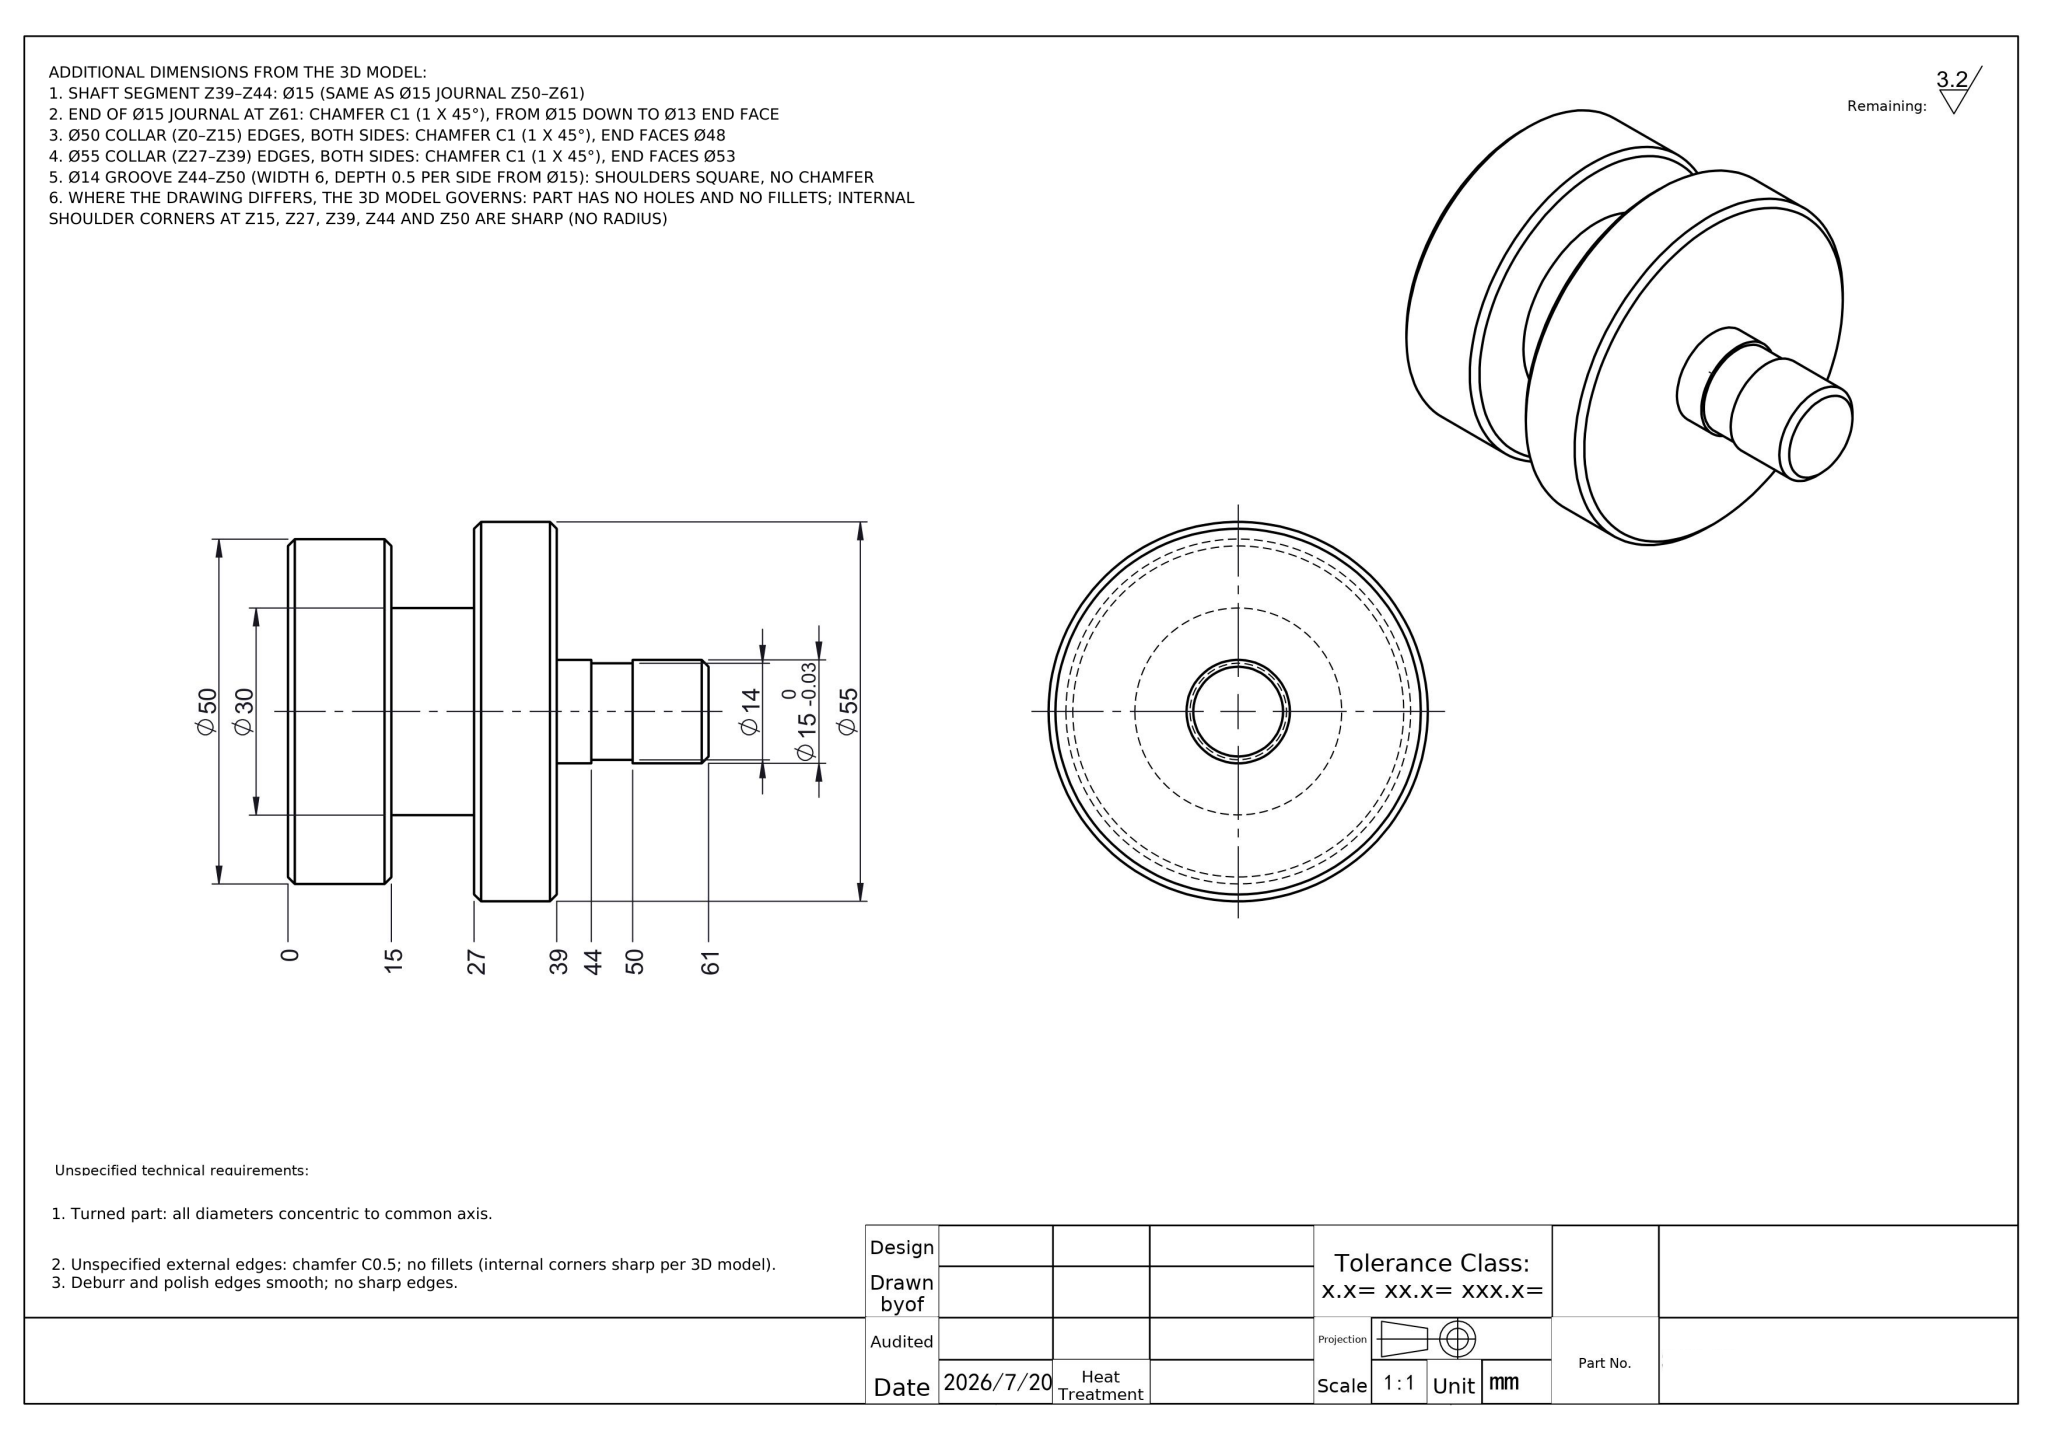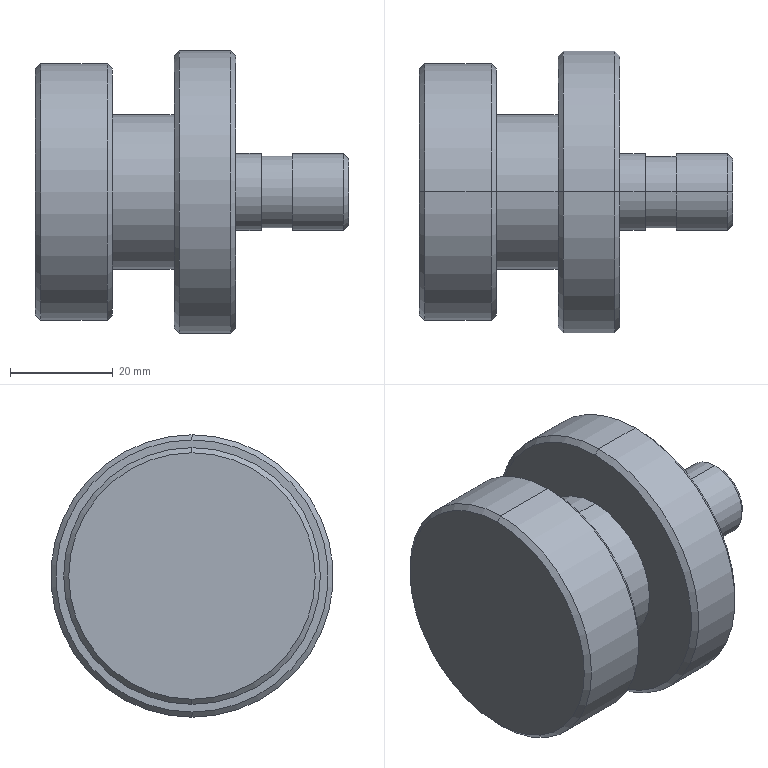Part | NX | mm | 1 solid | 29 faces | box 61 x 55 x 55 mm | volume 69848 mm3 | cylinder 12 | cone 10 | plane 7 | commonest cylinder face diameters 15 x4 14 x2 50 x2 30 x2 55 x2
STEP:
#1=CARTESIAN_POINT('',(39.,0.,-26.5));
#2=VERTEX_POINT('',#1);
#3=CARTESIAN_POINT('',(39.,0.,26.5));
#4=VERTEX_POINT('',#3);
#5=CARTESIAN_POINT('',(39.,0.,0.));
#6=DIRECTION('',(1.,0.,0.));
#7=DIRECTION('',(0.,0.,1.));
#8=AXIS2_PLACEMENT_3D('',#5,#6,#7);
#9=CIRCLE('',#8,26.5);
#10=EDGE_CURVE('',#2,#4,#9,.T.);
#11=ORIENTED_EDGE('',*,*,#10,.F.);
#12=CARTESIAN_POINT('',(38.,0.,-27.5));
#13=VERTEX_POINT('',#12);
#14=CARTESIAN_POINT('',(38.,0.,-27.5));
#15=DIRECTION('',(-0.7071,0.,-0.7071));
#16=VECTOR('',#15,1000.);
#17=LINE('',#14,#16);
#18=EDGE_CURVE('',#2,#13,#17,.T.);
#19=ORIENTED_EDGE('',*,*,#18,.T.);
#20=CARTESIAN_POINT('',(38.,0.,27.5));
#21=VERTEX_POINT('',#20);
#22=CARTESIAN_POINT('',(38.,0.,0.));
#23=DIRECTION('',(-1.,0.,0.));
#24=DIRECTION('',(0.,0.,1.));
#25=AXIS2_PLACEMENT_3D('',#22,#23,#24);
#26=CIRCLE('',#25,27.5);
#27=EDGE_CURVE('',#21,#13,#26,.T.);
#28=ORIENTED_EDGE('',*,*,#27,.F.);
#29=CARTESIAN_POINT('',(38.,0.,27.5));
#30=DIRECTION('',(-0.7071,0.,0.7071));
#31=VECTOR('',#30,1000.);
#32=LINE('',#29,#31);
#33=EDGE_CURVE('',#4,#21,#32,.T.);
#34=ORIENTED_EDGE('',*,*,#33,.F.);
#35=EDGE_LOOP('',(#11,#19,#28,#34));
#36=FACE_OUTER_BOUND('',#35,.T.);
#37=CARTESIAN_POINT('',(38.,0.,0.));
#38=DIRECTION('',(-1.,0.,0.));
#39=DIRECTION('',(0.,0.,1.));
#40=AXIS2_PLACEMENT_3D('',#37,#38,#39);
#41=CONICAL_SURFACE('',#40,27.5,0.7854);
#42=ADVANCED_FACE('',(#36),#41,.T.);
#43=CARTESIAN_POINT('',(61.,0.,-6.5));
#44=VERTEX_POINT('',#43);
#45=CARTESIAN_POINT('',(61.,0.,6.5));
#46=VERTEX_POINT('',#45);
#47=CARTESIAN_POINT('',(61.,0.,0.));
#48=DIRECTION('',(1.,0.,0.));
#49=DIRECTION('',(0.,0.,-1.));
#50=AXIS2_PLACEMENT_3D('',#47,#48,#49);
#51=CIRCLE('',#50,6.5);
#52=EDGE_CURVE('',#44,#46,#51,.T.);
#53=ORIENTED_EDGE('',*,*,#52,.F.);
#54=CARTESIAN_POINT('',(60.,0.,-7.5));
#55=VERTEX_POINT('',#54);
#56=CARTESIAN_POINT('',(61.,0.,-6.5));
#57=DIRECTION('',(-0.7071,0.,-0.7071));
#58=VECTOR('',#57,1000.);
#59=LINE('',#56,#58);
#60=EDGE_CURVE('',#44,#55,#59,.T.);
#61=ORIENTED_EDGE('',*,*,#60,.T.);
#62=CARTESIAN_POINT('',(60.,0.,7.5));
#63=VERTEX_POINT('',#62);
#64=CARTESIAN_POINT('',(60.,0.,0.));
#65=DIRECTION('',(-1.,0.,0.));
#66=DIRECTION('',(0.,0.,-1.));
#67=AXIS2_PLACEMENT_3D('',#64,#65,#66);
#68=CIRCLE('',#67,7.5);
#69=EDGE_CURVE('',#63,#55,#68,.T.);
#70=ORIENTED_EDGE('',*,*,#69,.F.);
#71=CARTESIAN_POINT('',(61.,0.,6.5));
#72=DIRECTION('',(-0.7071,0.,0.7071));
#73=VECTOR('',#72,1000.);
#74=LINE('',#71,#73);
#75=EDGE_CURVE('',#46,#63,#74,.T.);
#76=ORIENTED_EDGE('',*,*,#75,.F.);
#77=EDGE_LOOP('',(#53,#61,#70,#76));
#78=FACE_OUTER_BOUND('',#77,.T.);
#79=CARTESIAN_POINT('',(61.,0.,0.));
#80=DIRECTION('',(-1.,0.,0.));
#81=DIRECTION('',(0.,0.,1.));
#82=AXIS2_PLACEMENT_3D('',#79,#80,#81);
#83=CONICAL_SURFACE('',#82,6.5,0.7854);
#84=ADVANCED_FACE('',(#78),#83,.T.);
#85=ORIENTED_EDGE('',*,*,#69,.T.);
#86=CARTESIAN_POINT('',(50.,0.,-7.5));
#87=VERTEX_POINT('',#86);
#88=CARTESIAN_POINT('',(61.,0.,-7.5));
#89=DIRECTION('',(-1.,0.,0.));
#90=VECTOR('',#89,1000.);
#91=LINE('',#88,#90);
#92=EDGE_CURVE('',#55,#87,#91,.T.);
#93=ORIENTED_EDGE('',*,*,#92,.T.);
#94=CARTESIAN_POINT('',(50.,0.,7.5));
#95=VERTEX_POINT('',#94);
#96=CARTESIAN_POINT('',(50.,0.,0.));
#97=DIRECTION('',(1.,0.,0.));
#98=DIRECTION('',(0.,0.,-1.));
#99=AXIS2_PLACEMENT_3D('',#96,#97,#98);
#100=CIRCLE('',#99,7.5);
#101=EDGE_CURVE('',#87,#95,#100,.T.);
#102=ORIENTED_EDGE('',*,*,#101,.T.);
#103=CARTESIAN_POINT('',(61.,0.,7.5));
#104=DIRECTION('',(-1.,0.,0.));
#105=VECTOR('',#104,1000.);
#106=LINE('',#103,#105);
#107=EDGE_CURVE('',#63,#95,#106,.T.);
#108=ORIENTED_EDGE('',*,*,#107,.F.);
#109=EDGE_LOOP('',(#85,#93,#102,#108));
#110=FACE_OUTER_BOUND('',#109,.T.);
#111=CARTESIAN_POINT('',(61.,0.,0.));
#112=DIRECTION('',(-1.,0.,0.));
#113=DIRECTION('',(0.,0.,1.));
#114=AXIS2_PLACEMENT_3D('',#111,#112,#113);
#115=CYLINDRICAL_SURFACE('',#114,7.5);
#116=ADVANCED_FACE('',(#110),#115,.T.);
#117=CARTESIAN_POINT('',(50.,0.,-7.));
#118=VERTEX_POINT('',#117);
#119=CARTESIAN_POINT('',(50.,0.,7.));
#120=VERTEX_POINT('',#119);
#121=CARTESIAN_POINT('',(50.,0.,0.));
#122=DIRECTION('',(1.,0.,0.));
#123=DIRECTION('',(0.,0.,-1.));
#124=AXIS2_PLACEMENT_3D('',#121,#122,#123);
#125=CIRCLE('',#124,7.);
#126=EDGE_CURVE('',#118,#120,#125,.T.);
#127=ORIENTED_EDGE('',*,*,#126,.F.);
#128=CARTESIAN_POINT('',(44.,0.,-7.));
#129=VERTEX_POINT('',#128);
#130=CARTESIAN_POINT('',(50.,0.,-7.));
#131=DIRECTION('',(-1.,0.,0.));
#132=VECTOR('',#131,1000.);
#133=LINE('',#130,#132);
#134=EDGE_CURVE('',#118,#129,#133,.T.);
#135=ORIENTED_EDGE('',*,*,#134,.T.);
#136=CARTESIAN_POINT('',(44.,0.,7.));
#137=VERTEX_POINT('',#136);
#138=CARTESIAN_POINT('',(44.,0.,0.));
#139=DIRECTION('',(1.,0.,0.));
#140=DIRECTION('',(0.,0.,-1.));
#141=AXIS2_PLACEMENT_3D('',#138,#139,#140);
#142=CIRCLE('',#141,7.);
#143=EDGE_CURVE('',#129,#137,#142,.T.);
#144=ORIENTED_EDGE('',*,*,#143,.T.);
#145=CARTESIAN_POINT('',(50.,0.,7.));
#146=DIRECTION('',(-1.,0.,0.));
#147=VECTOR('',#146,1000.);
#148=LINE('',#145,#147);
#149=EDGE_CURVE('',#120,#137,#148,.T.);
#150=ORIENTED_EDGE('',*,*,#149,.F.);
#151=EDGE_LOOP('',(#127,#135,#144,#150));
#152=FACE_OUTER_BOUND('',#151,.T.);
#153=CARTESIAN_POINT('',(50.,0.,0.));
#154=DIRECTION('',(-1.,0.,0.));
#155=DIRECTION('',(0.,0.,1.));
#156=AXIS2_PLACEMENT_3D('',#153,#154,#155);
#157=CYLINDRICAL_SURFACE('',#156,7.);
#158=ADVANCED_FACE('',(#152),#157,.T.);
#159=CARTESIAN_POINT('',(27.,0.,26.5));
#160=VERTEX_POINT('',#159);
#161=CARTESIAN_POINT('',(27.,0.,-26.5));
#162=VERTEX_POINT('',#161);
#163=CARTESIAN_POINT('',(27.,0.,0.));
#164=DIRECTION('',(-1.,0.,0.));
#165=DIRECTION('',(0.,0.,-1.));
#166=AXIS2_PLACEMENT_3D('',#163,#164,#165);
#167=CIRCLE('',#166,26.5);
#168=EDGE_CURVE('',#160,#162,#167,.T.);
#169=ORIENTED_EDGE('',*,*,#168,.F.);
#170=CARTESIAN_POINT('',(28.,0.,27.5));
#171=VERTEX_POINT('',#170);
#172=CARTESIAN_POINT('',(27.,0.,26.5));
#173=DIRECTION('',(0.7071,0.,0.7071));
#174=VECTOR('',#173,1000.);
#175=LINE('',#172,#174);
#176=EDGE_CURVE('',#160,#171,#175,.T.);
#177=ORIENTED_EDGE('',*,*,#176,.T.);
#178=CARTESIAN_POINT('',(28.,0.,-27.5));
#179=VERTEX_POINT('',#178);
#180=CARTESIAN_POINT('',(28.,0.,0.));
#181=DIRECTION('',(1.,0.,0.));
#182=DIRECTION('',(0.,0.,-1.));
#183=AXIS2_PLACEMENT_3D('',#180,#181,#182);
#184=CIRCLE('',#183,27.5);
#185=EDGE_CURVE('',#179,#171,#184,.T.);
#186=ORIENTED_EDGE('',*,*,#185,.F.);
#187=CARTESIAN_POINT('',(27.,0.,-26.5));
#188=DIRECTION('',(0.7071,0.,-0.7071));
#189=VECTOR('',#188,1000.);
#190=LINE('',#187,#189);
#191=EDGE_CURVE('',#162,#179,#190,.T.);
#192=ORIENTED_EDGE('',*,*,#191,.F.);
#193=EDGE_LOOP('',(#169,#177,#186,#192));
#194=FACE_OUTER_BOUND('',#193,.T.);
#195=CARTESIAN_POINT('',(27.,0.,0.));
#196=DIRECTION('',(1.,0.,0.));
#197=DIRECTION('',(0.,0.,-1.));
#198=AXIS2_PLACEMENT_3D('',#195,#196,#197);
#199=CONICAL_SURFACE('',#198,26.5,0.7854);
#200=ADVANCED_FACE('',(#194),#199,.T.);
#201=CARTESIAN_POINT('',(-0.,0.,24.));
#202=VERTEX_POINT('',#201);
#203=CARTESIAN_POINT('',(-0.,0.,-24.));
#204=VERTEX_POINT('',#203);
#205=CARTESIAN_POINT('',(-0.,0.,0.));
#206=DIRECTION('',(-1.,0.,0.));
#207=DIRECTION('',(0.,0.,-1.));
#208=AXIS2_PLACEMENT_3D('',#205,#206,#207);
#209=CIRCLE('',#208,24.);
#210=EDGE_CURVE('',#202,#204,#209,.T.);
#211=ORIENTED_EDGE('',*,*,#210,.F.);
#212=CARTESIAN_POINT('',(1.,0.,25.));
#213=VERTEX_POINT('',#212);
#214=CARTESIAN_POINT('',(-0.,0.,24.));
#215=DIRECTION('',(0.7071,0.,0.7071));
#216=VECTOR('',#215,1000.);
#217=LINE('',#214,#216);
#218=EDGE_CURVE('',#202,#213,#217,.T.);
#219=ORIENTED_EDGE('',*,*,#218,.T.);
#220=CARTESIAN_POINT('',(1.,0.,-25.));
#221=VERTEX_POINT('',#220);
#222=CARTESIAN_POINT('',(1.,0.,0.));
#223=DIRECTION('',(1.,0.,0.));
#224=DIRECTION('',(0.,0.,-1.));
#225=AXIS2_PLACEMENT_3D('',#222,#223,#224);
#226=CIRCLE('',#225,25.);
#227=EDGE_CURVE('',#221,#213,#226,.T.);
#228=ORIENTED_EDGE('',*,*,#227,.F.);
#229=CARTESIAN_POINT('',(-0.,0.,-24.));
#230=DIRECTION('',(0.7071,0.,-0.7071));
#231=VECTOR('',#230,1000.);
#232=LINE('',#229,#231);
#233=EDGE_CURVE('',#204,#221,#232,.T.);
#234=ORIENTED_EDGE('',*,*,#233,.F.);
#235=EDGE_LOOP('',(#211,#219,#228,#234));
#236=FACE_OUTER_BOUND('',#235,.T.);
#237=CARTESIAN_POINT('',(-0.,0.,0.));
#238=DIRECTION('',(1.,0.,0.));
#239=DIRECTION('',(0.,0.,-1.));
#240=AXIS2_PLACEMENT_3D('',#237,#238,#239);
#241=CONICAL_SURFACE('',#240,24.,0.7854);
#242=ADVANCED_FACE('',(#236),#241,.T.);
#243=CARTESIAN_POINT('',(15.,0.,-24.));
#244=VERTEX_POINT('',#243);
#245=CARTESIAN_POINT('',(15.,0.,24.));
#246=VERTEX_POINT('',#245);
#247=CARTESIAN_POINT('',(15.,0.,0.));
#248=DIRECTION('',(1.,0.,0.));
#249=DIRECTION('',(0.,0.,1.));
#250=AXIS2_PLACEMENT_3D('',#247,#248,#249);
#251=CIRCLE('',#250,24.);
#252=EDGE_CURVE('',#244,#246,#251,.T.);
#253=ORIENTED_EDGE('',*,*,#252,.F.);
#254=CARTESIAN_POINT('',(14.,0.,-25.));
#255=VERTEX_POINT('',#254);
#256=CARTESIAN_POINT('',(14.,0.,-25.));
#257=DIRECTION('',(-0.7071,0.,-0.7071));
#258=VECTOR('',#257,1000.);
#259=LINE('',#256,#258);
#260=EDGE_CURVE('',#244,#255,#259,.T.);
#261=ORIENTED_EDGE('',*,*,#260,.T.);
#262=CARTESIAN_POINT('',(14.,0.,25.));
#263=VERTEX_POINT('',#262);
#264=CARTESIAN_POINT('',(14.,0.,0.));
#265=DIRECTION('',(-1.,0.,0.));
#266=DIRECTION('',(0.,0.,1.));
#267=AXIS2_PLACEMENT_3D('',#264,#265,#266);
#268=CIRCLE('',#267,25.);
#269=EDGE_CURVE('',#263,#255,#268,.T.);
#270=ORIENTED_EDGE('',*,*,#269,.F.);
#271=CARTESIAN_POINT('',(14.,0.,25.));
#272=DIRECTION('',(-0.7071,0.,0.7071));
#273=VECTOR('',#272,1000.);
#274=LINE('',#271,#273);
#275=EDGE_CURVE('',#246,#263,#274,.T.);
#276=ORIENTED_EDGE('',*,*,#275,.F.);
#277=EDGE_LOOP('',(#253,#261,#270,#276));
#278=FACE_OUTER_BOUND('',#277,.T.);
#279=CARTESIAN_POINT('',(14.,0.,0.));
#280=DIRECTION('',(-1.,0.,0.));
#281=DIRECTION('',(0.,0.,1.));
#282=AXIS2_PLACEMENT_3D('',#279,#280,#281);
#283=CONICAL_SURFACE('',#282,25.,0.7854);
#284=ADVANCED_FACE('',(#278),#283,.T.);
#285=ORIENTED_EDGE('',*,*,#269,.T.);
#286=CARTESIAN_POINT('',(0.,0.,-25.));
#287=DIRECTION('',(-1.,0.,0.));
#288=VECTOR('',#287,1000.);
#289=LINE('',#286,#288);
#290=EDGE_CURVE('',#255,#221,#289,.T.);
#291=ORIENTED_EDGE('',*,*,#290,.T.);
#292=ORIENTED_EDGE('',*,*,#227,.T.);
#293=CARTESIAN_POINT('',(0.,0.,25.));
#294=DIRECTION('',(-1.,0.,0.));
#295=VECTOR('',#294,1000.);
#296=LINE('',#293,#295);
#297=EDGE_CURVE('',#263,#213,#296,.T.);
#298=ORIENTED_EDGE('',*,*,#297,.F.);
#299=EDGE_LOOP('',(#285,#291,#292,#298));
#300=FACE_OUTER_BOUND('',#299,.T.);
#301=CARTESIAN_POINT('',(0.,0.,0.));
#302=DIRECTION('',(-1.,0.,0.));
#303=DIRECTION('',(0.,0.,1.));
#304=AXIS2_PLACEMENT_3D('',#301,#302,#303);
#305=CYLINDRICAL_SURFACE('',#304,25.);
#306=ADVANCED_FACE('',(#300),#305,.T.);
#307=CARTESIAN_POINT('',(27.,0.,15.));
#308=VERTEX_POINT('',#307);
#309=CARTESIAN_POINT('',(27.,0.,-15.));
#310=VERTEX_POINT('',#309);
#311=CARTESIAN_POINT('',(27.,0.,0.));
#312=DIRECTION('',(-1.,0.,0.));
#313=DIRECTION('',(0.,0.,1.));
#314=AXIS2_PLACEMENT_3D('',#311,#312,#313);
#315=CIRCLE('',#314,15.);
#316=EDGE_CURVE('',#308,#310,#315,.T.);
#317=ORIENTED_EDGE('',*,*,#316,.T.);
#318=CARTESIAN_POINT('',(15.,0.,-15.));
#319=VERTEX_POINT('',#318);
#320=CARTESIAN_POINT('',(0.,0.,-15.));
#321=DIRECTION('',(-1.,0.,0.));
#322=VECTOR('',#321,1000.);
#323=LINE('',#320,#322);
#324=EDGE_CURVE('',#310,#319,#323,.T.);
#325=ORIENTED_EDGE('',*,*,#324,.T.);
#326=CARTESIAN_POINT('',(15.,0.,15.));
#327=VERTEX_POINT('',#326);
#328=CARTESIAN_POINT('',(15.,0.,0.));
#329=DIRECTION('',(-1.,0.,0.));
#330=DIRECTION('',(0.,0.,1.));
#331=AXIS2_PLACEMENT_3D('',#328,#329,#330);
#332=CIRCLE('',#331,15.);
#333=EDGE_CURVE('',#327,#319,#332,.T.);
#334=ORIENTED_EDGE('',*,*,#333,.F.);
#335=CARTESIAN_POINT('',(0.,0.,15.));
#336=DIRECTION('',(-1.,0.,0.));
#337=VECTOR('',#336,1000.);
#338=LINE('',#335,#337);
#339=EDGE_CURVE('',#308,#327,#338,.T.);
#340=ORIENTED_EDGE('',*,*,#339,.F.);
#341=EDGE_LOOP('',(#317,#325,#334,#340));
#342=FACE_OUTER_BOUND('',#341,.T.);
#343=CARTESIAN_POINT('',(0.,0.,0.));
#344=DIRECTION('',(-1.,0.,0.));
#345=DIRECTION('',(0.,0.,1.));
#346=AXIS2_PLACEMENT_3D('',#343,#344,#345);
#347=CYLINDRICAL_SURFACE('',#346,15.);
#348=ADVANCED_FACE('',(#342),#347,.T.);
#349=ORIENTED_EDGE('',*,*,#27,.T.);
#350=CARTESIAN_POINT('',(0.,0.,-27.5));
#351=DIRECTION('',(-1.,0.,0.));
#352=VECTOR('',#351,1000.);
#353=LINE('',#350,#352);
#354=EDGE_CURVE('',#13,#179,#353,.T.);
#355=ORIENTED_EDGE('',*,*,#354,.T.);
#356=ORIENTED_EDGE('',*,*,#185,.T.);
#357=CARTESIAN_POINT('',(0.,0.,27.5));
#358=DIRECTION('',(-1.,0.,0.));
#359=VECTOR('',#358,1000.);
#360=LINE('',#357,#359);
#361=EDGE_CURVE('',#21,#171,#360,.T.);
#362=ORIENTED_EDGE('',*,*,#361,.F.);
#363=EDGE_LOOP('',(#349,#355,#356,#362));
#364=FACE_OUTER_BOUND('',#363,.T.);
#365=CARTESIAN_POINT('',(0.,0.,0.));
#366=DIRECTION('',(-1.,0.,0.));
#367=DIRECTION('',(0.,0.,1.));
#368=AXIS2_PLACEMENT_3D('',#365,#366,#367);
#369=CYLINDRICAL_SURFACE('',#368,27.5);
#370=ADVANCED_FACE('',(#364),#369,.T.);
#371=CARTESIAN_POINT('',(44.,0.,-7.5));
#372=VERTEX_POINT('',#371);
#373=CARTESIAN_POINT('',(44.,0.,7.5));
#374=VERTEX_POINT('',#373);
#375=CARTESIAN_POINT('',(44.,0.,0.));
#376=DIRECTION('',(1.,0.,0.));
#377=DIRECTION('',(0.,0.,-1.));
#378=AXIS2_PLACEMENT_3D('',#375,#376,#377);
#379=CIRCLE('',#378,7.5);
#380=EDGE_CURVE('',#372,#374,#379,.T.);
#381=ORIENTED_EDGE('',*,*,#380,.F.);
#382=CARTESIAN_POINT('',(39.,0.,-7.5));
#383=VERTEX_POINT('',#382);
#384=CARTESIAN_POINT('',(61.,0.,-7.5));
#385=DIRECTION('',(-1.,0.,0.));
#386=VECTOR('',#385,1000.);
#387=LINE('',#384,#386);
#388=EDGE_CURVE('',#372,#383,#387,.T.);
#389=ORIENTED_EDGE('',*,*,#388,.T.);
#390=CARTESIAN_POINT('',(39.,0.,7.5));
#391=VERTEX_POINT('',#390);
#392=CARTESIAN_POINT('',(39.,0.,0.));
#393=DIRECTION('',(1.,0.,0.));
#394=DIRECTION('',(0.,0.,1.));
#395=AXIS2_PLACEMENT_3D('',#392,#393,#394);
#396=CIRCLE('',#395,7.5);
#397=EDGE_CURVE('',#383,#391,#396,.T.);
#398=ORIENTED_EDGE('',*,*,#397,.T.);
#399=CARTESIAN_POINT('',(61.,0.,7.5));
#400=DIRECTION('',(-1.,0.,0.));
#401=VECTOR('',#400,1000.);
#402=LINE('',#399,#401);
#403=EDGE_CURVE('',#374,#391,#402,.T.);
#404=ORIENTED_EDGE('',*,*,#403,.F.);
#405=EDGE_LOOP('',(#381,#389,#398,#404));
#406=FACE_OUTER_BOUND('',#405,.T.);
#407=CARTESIAN_POINT('',(61.,0.,0.));
#408=DIRECTION('',(-1.,0.,0.));
#409=DIRECTION('',(0.,0.,1.));
#410=AXIS2_PLACEMENT_3D('',#407,#408,#409);
#411=CYLINDRICAL_SURFACE('',#410,7.5);
#412=ADVANCED_FACE('',(#406),#411,.T.);
#413=ORIENTED_EDGE('',*,*,#388,.F.);
#414=CARTESIAN_POINT('',(44.,0.,0.));
#415=DIRECTION('',(1.,0.,0.));
#416=DIRECTION('',(0.,0.,-1.));
#417=AXIS2_PLACEMENT_3D('',#414,#415,#416);
#418=CIRCLE('',#417,7.5);
#419=EDGE_CURVE('',#374,#372,#418,.T.);
#420=ORIENTED_EDGE('',*,*,#419,.F.);
#421=ORIENTED_EDGE('',*,*,#403,.T.);
#422=CARTESIAN_POINT('',(39.,0.,0.));
#423=DIRECTION('',(1.,0.,0.));
#424=DIRECTION('',(0.,0.,1.));
#425=AXIS2_PLACEMENT_3D('',#422,#423,#424);
#426=CIRCLE('',#425,7.5);
#427=EDGE_CURVE('',#391,#383,#426,.T.);
#428=ORIENTED_EDGE('',*,*,#427,.T.);
#429=EDGE_LOOP('',(#413,#420,#421,#428));
#430=FACE_OUTER_BOUND('',#429,.T.);
#431=CARTESIAN_POINT('',(61.,0.,0.));
#432=DIRECTION('',(-1.,0.,0.));
#433=DIRECTION('',(0.,0.,1.));
#434=AXIS2_PLACEMENT_3D('',#431,#432,#433);
#435=CYLINDRICAL_SURFACE('',#434,7.5);
#436=ADVANCED_FACE('',(#430),#435,.T.);
#437=CARTESIAN_POINT('',(39.,0.,0.));
#438=DIRECTION('',(1.,0.,0.));
#439=DIRECTION('',(0.,0.,1.));
#440=AXIS2_PLACEMENT_3D('',#437,#438,#439);
#441=CIRCLE('',#440,26.5);
#442=EDGE_CURVE('',#4,#2,#441,.T.);
#443=ORIENTED_EDGE('',*,*,#442,.T.);
#444=ORIENTED_EDGE('',*,*,#10,.T.);
#445=EDGE_LOOP('',(#443,#444));
#446=FACE_OUTER_BOUND('',#445,.T.);
#447=ORIENTED_EDGE('',*,*,#427,.F.);
#448=ORIENTED_EDGE('',*,*,#397,.F.);
#449=EDGE_LOOP('',(#447,#448));
#450=FACE_BOUND('',#449,.T.);
#451=CARTESIAN_POINT('',(39.,0.,0.));
#452=DIRECTION('',(-1.,0.,0.));
#453=DIRECTION('',(0.,0.,1.));
#454=AXIS2_PLACEMENT_3D('',#451,#452,#453);
#455=PLANE('',#454);
#456=ADVANCED_FACE('',(#446,#450),#455,.F.);
#457=CARTESIAN_POINT('',(-0.,0.,0.));
#458=DIRECTION('',(-1.,0.,0.));
#459=DIRECTION('',(0.,0.,-1.));
#460=AXIS2_PLACEMENT_3D('',#457,#458,#459);
#461=CIRCLE('',#460,24.);
#462=EDGE_CURVE('',#204,#202,#461,.T.);
#463=ORIENTED_EDGE('',*,*,#462,.T.);
#464=ORIENTED_EDGE('',*,*,#210,.T.);
#465=EDGE_LOOP('',(#463,#464));
#466=FACE_OUTER_BOUND('',#465,.T.);
#467=CARTESIAN_POINT('',(-0.,25.,0.));
#468=DIRECTION('',(1.,0.,0.));
#469=DIRECTION('',(0.,0.,-1.));
#470=AXIS2_PLACEMENT_3D('',#467,#468,#469);
#471=PLANE('',#470);
#472=ADVANCED_FACE('',(#466),#471,.F.);
#473=ORIENTED_EDGE('',*,*,#354,.F.);
#474=CARTESIAN_POINT('',(38.,0.,0.));
#475=DIRECTION('',(-1.,0.,0.));
#476=DIRECTION('',(0.,0.,1.));
#477=AXIS2_PLACEMENT_3D('',#474,#475,#476);
#478=CIRCLE('',#477,27.5);
#479=EDGE_CURVE('',#13,#21,#478,.T.);
#480=ORIENTED_EDGE('',*,*,#479,.T.);
#481=ORIENTED_EDGE('',*,*,#361,.T.);
#482=CARTESIAN_POINT('',(28.,0.,0.));
#483=DIRECTION('',(1.,0.,0.));
#484=DIRECTION('',(0.,0.,-1.));
#485=AXIS2_PLACEMENT_3D('',#482,#483,#484);
#486=CIRCLE('',#485,27.5);
#487=EDGE_CURVE('',#171,#179,#486,.T.);
#488=ORIENTED_EDGE('',*,*,#487,.T.);
#489=EDGE_LOOP('',(#473,#480,#481,#488));
#490=FACE_OUTER_BOUND('',#489,.T.);
#491=CARTESIAN_POINT('',(0.,0.,0.));
#492=DIRECTION('',(-1.,0.,0.));
#493=DIRECTION('',(0.,0.,1.));
#494=AXIS2_PLACEMENT_3D('',#491,#492,#493);
#495=CYLINDRICAL_SURFACE('',#494,27.5);
#496=ADVANCED_FACE('',(#490),#495,.T.);
#497=CARTESIAN_POINT('',(27.,0.,0.));
#498=DIRECTION('',(-1.,0.,0.));
#499=DIRECTION('',(0.,0.,-1.));
#500=AXIS2_PLACEMENT_3D('',#497,#498,#499);
#501=CIRCLE('',#500,26.5);
#502=EDGE_CURVE('',#162,#160,#501,.T.);
#503=ORIENTED_EDGE('',*,*,#502,.T.);
#504=ORIENTED_EDGE('',*,*,#168,.T.);
#505=EDGE_LOOP('',(#503,#504));
#506=FACE_OUTER_BOUND('',#505,.T.);
#507=ORIENTED_EDGE('',*,*,#316,.F.);
#508=CARTESIAN_POINT('',(27.,0.,0.));
#509=DIRECTION('',(-1.,0.,0.));
#510=DIRECTION('',(0.,0.,1.));
#511=AXIS2_PLACEMENT_3D('',#508,#509,#510);
#512=CIRCLE('',#511,15.);
#513=EDGE_CURVE('',#310,#308,#512,.T.);
#514=ORIENTED_EDGE('',*,*,#513,.F.);
#515=EDGE_LOOP('',(#507,#514));
#516=FACE_BOUND('',#515,.T.);
#517=CARTESIAN_POINT('',(27.,27.5,0.));
#518=DIRECTION('',(1.,0.,0.));
#519=DIRECTION('',(0.,0.,-1.));
#520=AXIS2_PLACEMENT_3D('',#517,#518,#519);
#521=PLANE('',#520);
#522=ADVANCED_FACE('',(#506,#516),#521,.F.);
#523=ORIENTED_EDGE('',*,*,#324,.F.);
#524=ORIENTED_EDGE('',*,*,#513,.T.);
#525=ORIENTED_EDGE('',*,*,#339,.T.);
#526=CARTESIAN_POINT('',(15.,0.,0.));
#527=DIRECTION('',(-1.,0.,0.));
#528=DIRECTION('',(0.,0.,1.));
#529=AXIS2_PLACEMENT_3D('',#526,#527,#528);
#530=CIRCLE('',#529,15.);
#531=EDGE_CURVE('',#319,#327,#530,.T.);
#532=ORIENTED_EDGE('',*,*,#531,.F.);
#533=EDGE_LOOP('',(#523,#524,#525,#532));
#534=FACE_OUTER_BOUND('',#533,.T.);
#535=CARTESIAN_POINT('',(0.,0.,0.));
#536=DIRECTION('',(-1.,0.,0.));
#537=DIRECTION('',(0.,0.,1.));
#538=AXIS2_PLACEMENT_3D('',#535,#536,#537);
#539=CYLINDRICAL_SURFACE('',#538,15.);
#540=ADVANCED_FACE('',(#534),#539,.T.);
#541=CARTESIAN_POINT('',(15.,0.,0.));
#542=DIRECTION('',(1.,0.,0.));
#543=DIRECTION('',(0.,0.,1.));
#544=AXIS2_PLACEMENT_3D('',#541,#542,#543);
#545=CIRCLE('',#544,24.);
#546=EDGE_CURVE('',#246,#244,#545,.T.);
#547=ORIENTED_EDGE('',*,*,#546,.T.);
#548=ORIENTED_EDGE('',*,*,#252,.T.);
#549=EDGE_LOOP('',(#547,#548));
#550=FACE_OUTER_BOUND('',#549,.T.);
#551=ORIENTED_EDGE('',*,*,#333,.T.);
#552=ORIENTED_EDGE('',*,*,#531,.T.);
#553=EDGE_LOOP('',(#551,#552));
#554=FACE_BOUND('',#553,.T.);
#555=CARTESIAN_POINT('',(15.,15.,0.));
#556=DIRECTION('',(-1.,0.,0.));
#557=DIRECTION('',(0.,0.,1.));
#558=AXIS2_PLACEMENT_3D('',#555,#556,#557);
#559=PLANE('',#558);
#560=ADVANCED_FACE('',(#550,#554),#559,.F.);
#561=ORIENTED_EDGE('',*,*,#290,.F.);
#562=CARTESIAN_POINT('',(14.,0.,0.));
#563=DIRECTION('',(-1.,0.,0.));
#564=DIRECTION('',(0.,0.,1.));
#565=AXIS2_PLACEMENT_3D('',#562,#563,#564);
#566=CIRCLE('',#565,25.);
#567=EDGE_CURVE('',#255,#263,#566,.T.);
#568=ORIENTED_EDGE('',*,*,#567,.T.);
#569=ORIENTED_EDGE('',*,*,#297,.T.);
#570=CARTESIAN_POINT('',(1.,0.,0.));
#571=DIRECTION('',(1.,0.,0.));
#572=DIRECTION('',(0.,0.,-1.));
#573=AXIS2_PLACEMENT_3D('',#570,#571,#572);
#574=CIRCLE('',#573,25.);
#575=EDGE_CURVE('',#213,#221,#574,.T.);
#576=ORIENTED_EDGE('',*,*,#575,.T.);
#577=EDGE_LOOP('',(#561,#568,#569,#576));
#578=FACE_OUTER_BOUND('',#577,.T.);
#579=CARTESIAN_POINT('',(0.,0.,0.));
#580=DIRECTION('',(-1.,0.,0.));
#581=DIRECTION('',(0.,0.,1.));
#582=AXIS2_PLACEMENT_3D('',#579,#580,#581);
#583=CYLINDRICAL_SURFACE('',#582,25.);
#584=ADVANCED_FACE('',(#578),#583,.T.);
#585=ORIENTED_EDGE('',*,*,#260,.F.);
#586=ORIENTED_EDGE('',*,*,#546,.F.);
#587=ORIENTED_EDGE('',*,*,#275,.T.);
#588=ORIENTED_EDGE('',*,*,#567,.F.);
#589=EDGE_LOOP('',(#585,#586,#587,#588));
#590=FACE_OUTER_BOUND('',#589,.T.);
#591=CARTESIAN_POINT('',(14.,0.,0.));
#592=DIRECTION('',(-1.,0.,0.));
#593=DIRECTION('',(0.,0.,1.));
#594=AXIS2_PLACEMENT_3D('',#591,#592,#593);
#595=CONICAL_SURFACE('',#594,25.,0.7854);
#596=ADVANCED_FACE('',(#590),#595,.T.);
#597=ORIENTED_EDGE('',*,*,#218,.F.);
#598=ORIENTED_EDGE('',*,*,#462,.F.);
#599=ORIENTED_EDGE('',*,*,#233,.T.);
#600=ORIENTED_EDGE('',*,*,#575,.F.);
#601=EDGE_LOOP('',(#597,#598,#599,#600));
#602=FACE_OUTER_BOUND('',#601,.T.);
#603=CARTESIAN_POINT('',(-0.,0.,0.));
#604=DIRECTION('',(1.,0.,0.));
#605=DIRECTION('',(0.,0.,-1.));
#606=AXIS2_PLACEMENT_3D('',#603,#604,#605);
#607=CONICAL_SURFACE('',#606,24.,0.7854);
#608=ADVANCED_FACE('',(#602),#607,.T.);
#609=ORIENTED_EDGE('',*,*,#176,.F.);
#610=ORIENTED_EDGE('',*,*,#502,.F.);
#611=ORIENTED_EDGE('',*,*,#191,.T.);
#612=ORIENTED_EDGE('',*,*,#487,.F.);
#613=EDGE_LOOP('',(#609,#610,#611,#612));
#614=FACE_OUTER_BOUND('',#613,.T.);
#615=CARTESIAN_POINT('',(27.,0.,0.));
#616=DIRECTION('',(1.,0.,0.));
#617=DIRECTION('',(0.,0.,-1.));
#618=AXIS2_PLACEMENT_3D('',#615,#616,#617);
#619=CONICAL_SURFACE('',#618,26.5,0.7854);
#620=ADVANCED_FACE('',(#614),#619,.T.);
#621=CARTESIAN_POINT('',(50.,0.,0.));
#622=DIRECTION('',(1.,0.,0.));
#623=DIRECTION('',(0.,0.,-1.));
#624=AXIS2_PLACEMENT_3D('',#621,#622,#623);
#625=CIRCLE('',#624,7.);
#626=EDGE_CURVE('',#120,#118,#625,.T.);
#627=ORIENTED_EDGE('',*,*,#626,.T.);
#628=ORIENTED_EDGE('',*,*,#126,.T.);
#629=EDGE_LOOP('',(#627,#628));
#630=FACE_BOUND('',#629,.T.);
#631=CARTESIAN_POINT('',(50.,0.,0.));
#632=DIRECTION('',(1.,0.,0.));
#633=DIRECTION('',(0.,0.,-1.));
#634=AXIS2_PLACEMENT_3D('',#631,#632,#633);
#635=CIRCLE('',#634,7.5);
#636=EDGE_CURVE('',#95,#87,#635,.T.);
#637=ORIENTED_EDGE('',*,*,#636,.F.);
#638=ORIENTED_EDGE('',*,*,#101,.F.);
#639=EDGE_LOOP('',(#637,#638));
#640=FACE_OUTER_BOUND('',#639,.T.);
#641=CARTESIAN_POINT('',(50.,0.,0.));
#642=DIRECTION('',(1.,0.,0.));
#643=DIRECTION('',(0.,0.,-1.));
#644=AXIS2_PLACEMENT_3D('',#641,#642,#643);
#645=PLANE('',#644);
#646=ADVANCED_FACE('',(#630,#640),#645,.F.);
#647=CARTESIAN_POINT('',(44.,0.,0.));
#648=DIRECTION('',(1.,0.,0.));
#649=DIRECTION('',(0.,0.,-1.));
#650=AXIS2_PLACEMENT_3D('',#647,#648,#649);
#651=CIRCLE('',#650,7.);
#652=EDGE_CURVE('',#137,#129,#651,.T.);
#653=ORIENTED_EDGE('',*,*,#652,.F.);
#654=ORIENTED_EDGE('',*,*,#143,.F.);
#655=EDGE_LOOP('',(#653,#654));
#656=FACE_BOUND('',#655,.T.);
#657=ORIENTED_EDGE('',*,*,#419,.T.);
#658=ORIENTED_EDGE('',*,*,#380,.T.);
#659=EDGE_LOOP('',(#657,#658));
#660=FACE_OUTER_BOUND('',#659,.T.);
#661=CARTESIAN_POINT('',(44.,0.,0.));
#662=DIRECTION('',(1.,0.,0.));
#663=DIRECTION('',(0.,0.,-1.));
#664=AXIS2_PLACEMENT_3D('',#661,#662,#663);
#665=PLANE('',#664);
#666=ADVANCED_FACE('',(#656,#660),#665,.T.);
#667=ORIENTED_EDGE('',*,*,#134,.F.);
#668=ORIENTED_EDGE('',*,*,#626,.F.);
#669=ORIENTED_EDGE('',*,*,#149,.T.);
#670=ORIENTED_EDGE('',*,*,#652,.T.);
#671=EDGE_LOOP('',(#667,#668,#669,#670));
#672=FACE_OUTER_BOUND('',#671,.T.);
#673=CARTESIAN_POINT('',(50.,0.,0.));
#674=DIRECTION('',(-1.,0.,0.));
#675=DIRECTION('',(0.,0.,1.));
#676=AXIS2_PLACEMENT_3D('',#673,#674,#675);
#677=CYLINDRICAL_SURFACE('',#676,7.);
#678=ADVANCED_FACE('',(#672),#677,.T.);
#679=CARTESIAN_POINT('',(61.,0.,0.));
#680=DIRECTION('',(1.,0.,0.));
#681=DIRECTION('',(0.,0.,-1.));
#682=AXIS2_PLACEMENT_3D('',#679,#680,#681);
#683=CIRCLE('',#682,6.5);
#684=EDGE_CURVE('',#46,#44,#683,.T.);
#685=ORIENTED_EDGE('',*,*,#684,.T.);
#686=ORIENTED_EDGE('',*,*,#52,.T.);
#687=EDGE_LOOP('',(#685,#686));
#688=FACE_OUTER_BOUND('',#687,.T.);
#689=CARTESIAN_POINT('',(61.,0.,0.));
#690=DIRECTION('',(1.,0.,0.));
#691=DIRECTION('',(0.,0.,-1.));
#692=AXIS2_PLACEMENT_3D('',#689,#690,#691);
#693=PLANE('',#692);
#694=ADVANCED_FACE('',(#688),#693,.T.);
#695=ORIENTED_EDGE('',*,*,#92,.F.);
#696=CARTESIAN_POINT('',(60.,0.,0.));
#697=DIRECTION('',(-1.,0.,0.));
#698=DIRECTION('',(0.,0.,-1.));
#699=AXIS2_PLACEMENT_3D('',#696,#697,#698);
#700=CIRCLE('',#699,7.5);
#701=EDGE_CURVE('',#55,#63,#700,.T.);
#702=ORIENTED_EDGE('',*,*,#701,.T.);
#703=ORIENTED_EDGE('',*,*,#107,.T.);
#704=ORIENTED_EDGE('',*,*,#636,.T.);
#705=EDGE_LOOP('',(#695,#702,#703,#704));
#706=FACE_OUTER_BOUND('',#705,.T.);
#707=CARTESIAN_POINT('',(61.,0.,0.));
#708=DIRECTION('',(-1.,0.,0.));
#709=DIRECTION('',(0.,0.,1.));
#710=AXIS2_PLACEMENT_3D('',#707,#708,#709);
#711=CYLINDRICAL_SURFACE('',#710,7.5);
#712=ADVANCED_FACE('',(#706),#711,.T.);
#713=ORIENTED_EDGE('',*,*,#60,.F.);
#714=ORIENTED_EDGE('',*,*,#684,.F.);
#715=ORIENTED_EDGE('',*,*,#75,.T.);
#716=ORIENTED_EDGE('',*,*,#701,.F.);
#717=EDGE_LOOP('',(#713,#714,#715,#716));
#718=FACE_OUTER_BOUND('',#717,.T.);
#719=CARTESIAN_POINT('',(61.,0.,0.));
#720=DIRECTION('',(-1.,0.,0.));
#721=DIRECTION('',(0.,0.,1.));
#722=AXIS2_PLACEMENT_3D('',#719,#720,#721);
#723=CONICAL_SURFACE('',#722,6.5,0.7854);
#724=ADVANCED_FACE('',(#718),#723,.T.);
#725=ORIENTED_EDGE('',*,*,#18,.F.);
#726=ORIENTED_EDGE('',*,*,#442,.F.);
#727=ORIENTED_EDGE('',*,*,#33,.T.);
#728=ORIENTED_EDGE('',*,*,#479,.F.);
#729=EDGE_LOOP('',(#725,#726,#727,#728));
#730=FACE_OUTER_BOUND('',#729,.T.);
#731=CARTESIAN_POINT('',(38.,0.,0.));
#732=DIRECTION('',(-1.,0.,0.));
#733=DIRECTION('',(0.,0.,1.));
#734=AXIS2_PLACEMENT_3D('',#731,#732,#733);
#735=CONICAL_SURFACE('',#734,27.5,0.7854);
#736=ADVANCED_FACE('',(#730),#735,.T.);
#737=CLOSED_SHELL('',(#42,#84,#116,#158,#200,#242,#284,#306,#348,#370,#412,#436,#456,#472,#496,#522,#540,#560,#584,#596,#608,#620,#646,#666,#678,#694,#712,#724,#736));
#738=MANIFOLD_SOLID_BREP('',#737);
#739=CARTESIAN_POINT('',(0.,0.,0.));
#740=DIRECTION('',(0.,0.,1.));
#741=DIRECTION('',(1.,0.,0.));
#742=AXIS2_PLACEMENT_3D('',#739,#740,#741);
#743=(LENGTH_UNIT()NAMED_UNIT(*)SI_UNIT(.MILLI.,.METRE.));
#744=UNCERTAINTY_MEASURE_WITH_UNIT(LENGTH_MEASURE(0.00001),#743,'','');
#745=(NAMED_UNIT(*)PLANE_ANGLE_UNIT()SI_UNIT($,.RADIAN.));
#746=(NAMED_UNIT(*)SI_UNIT($,.STERADIAN.)SOLID_ANGLE_UNIT());
#747=(GEOMETRIC_REPRESENTATION_CONTEXT(3)GLOBAL_UNCERTAINTY_ASSIGNED_CONTEXT((#744))GLOBAL_UNIT_ASSIGNED_CONTEXT((#743,#745,#746))REPRESENTATION_CONTEXT('',''));
#748=ADVANCED_BREP_SHAPE_REPRESENTATION('',(#738,#742),#747);
#749=COLOUR_RGB('',0.7922,0.8196,0.9333);
#750=FILL_AREA_STYLE_COLOUR('',#749);
#751=FILL_AREA_STYLE('',(#750));
#752=SURFACE_STYLE_FILL_AREA(#751);
#753=SURFACE_SIDE_STYLE('',(#752));
#754=SURFACE_STYLE_USAGE(.BOTH.,#753);
#755=PRESENTATION_STYLE_ASSIGNMENT((#754));
#756=STYLED_ITEM('',(#755),#738);
#757=(LENGTH_UNIT()NAMED_UNIT(*)SI_UNIT(.MILLI.,.METRE.));
#758=UNCERTAINTY_MEASURE_WITH_UNIT(LENGTH_MEASURE(0.00001),#757,'','');
#759=(NAMED_UNIT(*)PLANE_ANGLE_UNIT()SI_UNIT($,.RADIAN.));
#760=(NAMED_UNIT(*)SI_UNIT($,.STERADIAN.)SOLID_ANGLE_UNIT());
#761=(GEOMETRIC_REPRESENTATION_CONTEXT(3)GLOBAL_UNCERTAINTY_ASSIGNED_CONTEXT((#758))GLOBAL_UNIT_ASSIGNED_CONTEXT((#757,#759,#760))REPRESENTATION_CONTEXT('',''));
#762=MECHANICAL_DESIGN_GEOMETRIC_PRESENTATION_REPRESENTATION('',(#756),#761);
#763=PRESENTATION_LAYER_ASSIGNMENT('','',(#756));